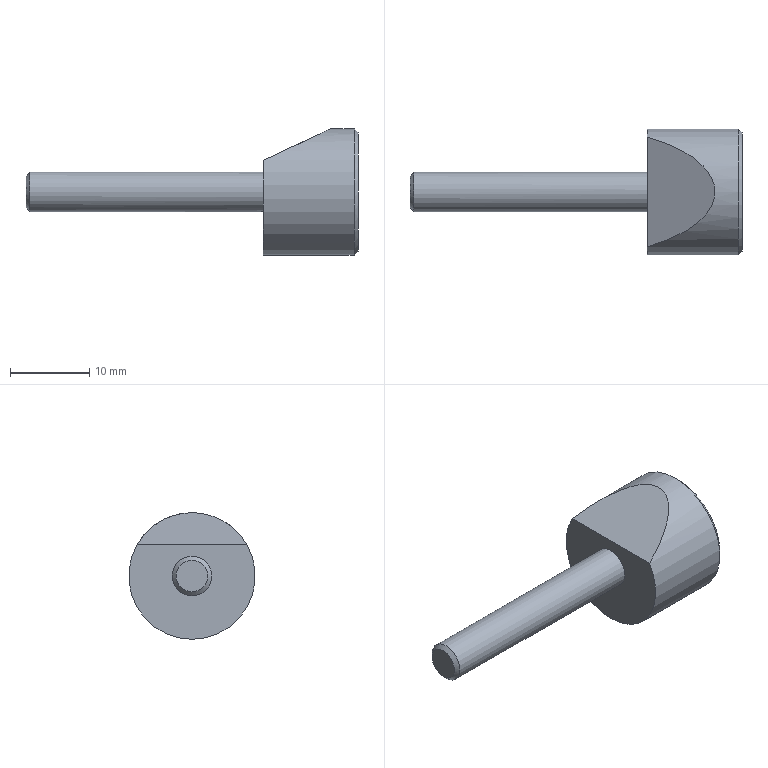Component | NX | LOCKING_SHAFT | 1 solid | 8 faces | box 42 x 16 x 16 mm | volume 2856 mm3 | plane 4 | cylinder 2 | cone 2 | commonest cylinder face diameters 16 x1 5 x1
STEP:
#1=CARTESIAN_POINT('',(0.,0.,0.));
#2=DIRECTION('',(0.,0.,1.));
#3=DIRECTION('',(1.,0.,0.));
#4=AXIS2_PLACEMENT_3D('',#1,#2,#3);
#5=CARTESIAN_POINT('',(109.666,163.398,144.15));
#6=VERTEX_POINT('',#5);
#7=CARTESIAN_POINT('',(109.666,170.327,156.15));
#8=VERTEX_POINT('',#7);
#9=CARTESIAN_POINT('',(109.666,163.398,152.15));
#10=DIRECTION('',(-1.,0.,0.));
#11=DIRECTION('',(0.,0.,-1.));
#12=AXIS2_PLACEMENT_3D('',#9,#10,#11);
#13=CIRCLE('',#12,8.);
#14=CARTESIAN_POINT('',(98.166,163.398,152.15));
#15=DIRECTION('',(1.,0.,0.));
#16=DIRECTION('',(0.,0.,1.));
#17=AXIS2_PLACEMENT_3D('',#14,#15,#16);
#18=CYLINDRICAL_SURFACE('',#17,8.);
#19=CARTESIAN_POINT('',(9.425,11.5));
#20=DIRECTION('',(-1.,0.));
#21=VECTOR('',#20,1.);
#22=LINE('',#19,#21);
#23=(GEOMETRIC_REPRESENTATION_CONTEXT(2)PARAMETRIC_REPRESENTATION_CONTEXT()REPRESENTATION_CONTEXT('',''));
#24=DEFINITIONAL_REPRESENTATION('',(#22),#23);
#25=PCURVE('',#18,#24);
#26=CARTESIAN_POINT('',(109.666,163.398,152.15));
#27=DIRECTION('',(-1.,0.,0.));
#28=DIRECTION('',(0.,0.,-1.));
#29=AXIS2_PLACEMENT_3D('',#26,#27,#28);
#30=CONICAL_SURFACE('',#29,8.,0.7854);
#31=CARTESIAN_POINT('',(0.,0.));
#32=DIRECTION('',(1.,0.));
#33=VECTOR('',#32,1.);
#34=LINE('',#31,#33);
#35=(GEOMETRIC_REPRESENTATION_CONTEXT(2)PARAMETRIC_REPRESENTATION_CONTEXT()REPRESENTATION_CONTEXT('',''));
#36=DEFINITIONAL_REPRESENTATION('',(#34),#35);
#37=PCURVE('',#30,#36);
#38=SURFACE_CURVE('',#13,(#25,#37),.PCURVE_S1.);
#39=EDGE_CURVE('',#6,#8,#38,.T.);
#40=ORIENTED_EDGE('',*,*,#39,.T.);
#41=CARTESIAN_POINT('',(98.166,170.327,156.15));
#42=VERTEX_POINT('',#41);
#43=CARTESIAN_POINT('',(98.166,170.327,156.15));
#44=CARTESIAN_POINT('',(109.666,170.327,156.15));
#45=B_SPLINE_CURVE_WITH_KNOTS('',1,(#43,#44),.UNSPECIFIED.,.F.,.F.,(2,2),(0.,11.5),.PIECEWISE_BEZIER_KNOTS.);
#46=CARTESIAN_POINT('',(5.236,0.));
#47=DIRECTION('',(0.,1.));
#48=VECTOR('',#47,1.);
#49=LINE('',#46,#48);
#50=(GEOMETRIC_REPRESENTATION_CONTEXT(2)PARAMETRIC_REPRESENTATION_CONTEXT()REPRESENTATION_CONTEXT('',''));
#51=DEFINITIONAL_REPRESENTATION('',(#49),#50);
#52=PCURVE('',#18,#51);
#53=CARTESIAN_POINT('',(11.519,0.));
#54=DIRECTION('',(0.,1.));
#55=VECTOR('',#54,1.);
#56=LINE('',#53,#55);
#57=(GEOMETRIC_REPRESENTATION_CONTEXT(2)PARAMETRIC_REPRESENTATION_CONTEXT()REPRESENTATION_CONTEXT('',''));
#58=DEFINITIONAL_REPRESENTATION('',(#56),#57);
#59=PCURVE('',#18,#58);
#60=SEAM_CURVE('',#45,(#52,#59),.PCURVE_S1.);
#61=EDGE_CURVE('',#42,#8,#60,.T.);
#62=ORIENTED_EDGE('',*,*,#61,.F.);
#63=CARTESIAN_POINT('',(98.166,156.47,156.15));
#64=VERTEX_POINT('',#63);
#65=CARTESIAN_POINT('',(89.588,163.398,152.15));
#66=DIRECTION('',(-0.4226,0.,0.9063));
#67=DIRECTION('',(0.9063,0.,0.4226));
#68=AXIS2_PLACEMENT_3D('',#65,#66,#67);
#69=ELLIPSE('',#68,18.93,8.);
#70=CARTESIAN_POINT('',(7.33,-0.));
#71=CARTESIAN_POINT('',(7.299,0.4715));
#72=CARTESIAN_POINT('',(7.235,1.388));
#73=CARTESIAN_POINT('',(7.14,2.674));
#74=CARTESIAN_POINT('',(7.045,3.857));
#75=CARTESIAN_POINT('',(6.95,4.928));
#76=CARTESIAN_POINT('',(6.854,5.876));
#77=CARTESIAN_POINT('',(6.759,6.694));
#78=CARTESIAN_POINT('',(6.664,7.373));
#79=CARTESIAN_POINT('',(6.569,7.908));
#80=CARTESIAN_POINT('',(6.474,8.293));
#81=CARTESIAN_POINT('',(6.378,8.526));
#82=CARTESIAN_POINT('',(6.283,8.604));
#83=CARTESIAN_POINT('',(6.188,8.526));
#84=CARTESIAN_POINT('',(6.093,8.293));
#85=CARTESIAN_POINT('',(5.998,7.908));
#86=CARTESIAN_POINT('',(5.902,7.373));
#87=CARTESIAN_POINT('',(5.807,6.694));
#88=CARTESIAN_POINT('',(5.712,5.876));
#89=CARTESIAN_POINT('',(5.617,4.928));
#90=CARTESIAN_POINT('',(5.522,3.857));
#91=CARTESIAN_POINT('',(5.426,2.674));
#92=CARTESIAN_POINT('',(5.331,1.388));
#93=CARTESIAN_POINT('',(5.268,0.4715));
#94=CARTESIAN_POINT('',(5.236,0.));
#95=B_SPLINE_CURVE_WITH_KNOTS('',3,(#70,#71,#72,#73,#74,#75,#76,#77,#78,#79,#80,#81,#82,#83,#84,#85,#86,#87,#88,#89,#90,#91,#92,#93,#94),.UNSPECIFIED.,.F.,.F.,(4,1,1,1,1,1,1,1,1,1,1,1,1,1,1,1,1,1,1,1,1,1,4),(5.236,5.331,5.426,5.522,5.617,5.712,5.807,5.902,5.998,6.093,6.188,6.283,6.378,6.474,6.569,6.664,6.759,6.854,6.95,7.045,7.14,7.235,7.33),.QUASI_UNIFORM_KNOTS.);
#96=(GEOMETRIC_REPRESENTATION_CONTEXT(2)PARAMETRIC_REPRESENTATION_CONTEXT()REPRESENTATION_CONTEXT('',''));
#97=DEFINITIONAL_REPRESENTATION('',(#95),#96);
#98=PCURVE('',#18,#97);
#99=CARTESIAN_POINT('',(98.166,133.398,156.15));
#100=DIRECTION('',(-0.4226,0.,0.9063));
#101=DIRECTION('',(-0.9063,0.,-0.4226));
#102=AXIS2_PLACEMENT_3D('',#99,#100,#101);
#103=PLANE('',#102);
#104=CARTESIAN_POINT('',(9.465,-30.));
#105=DIRECTION('',(-1.,0.));
#106=AXIS2_PLACEMENT_2D('',#104,#105);
#107=ELLIPSE('',#106,18.93,8.);
#108=(GEOMETRIC_REPRESENTATION_CONTEXT(2)PARAMETRIC_REPRESENTATION_CONTEXT()REPRESENTATION_CONTEXT('',''));
#109=DEFINITIONAL_REPRESENTATION('',(#107),#108);
#110=PCURVE('',#103,#109);
#111=SURFACE_CURVE('',#69,(#98,#110),.PCURVE_S1.);
#112=EDGE_CURVE('',#64,#42,#111,.T.);
#113=ORIENTED_EDGE('',*,*,#112,.F.);
#114=CARTESIAN_POINT('',(98.166,163.398,152.15));
#115=DIRECTION('',(-1.,0.,0.));
#116=DIRECTION('',(0.,-1.,0.));
#117=AXIS2_PLACEMENT_3D('',#114,#115,#116);
#118=CIRCLE('',#117,8.);
#119=CARTESIAN_POINT('',(14.137,0.));
#120=DIRECTION('',(-1.,0.));
#121=VECTOR('',#120,1.);
#122=LINE('',#119,#121);
#123=(GEOMETRIC_REPRESENTATION_CONTEXT(2)PARAMETRIC_REPRESENTATION_CONTEXT()REPRESENTATION_CONTEXT('',''));
#124=DEFINITIONAL_REPRESENTATION('',(#122),#123);
#125=PCURVE('',#18,#124);
#126=CARTESIAN_POINT('',(98.166,163.398,152.15));
#127=DIRECTION('',(-1.,0.,0.));
#128=DIRECTION('',(0.,0.,-1.));
#129=AXIS2_PLACEMENT_3D('',#126,#127,#128);
#130=PLANE('',#129);
#131=CARTESIAN_POINT('',(0.,0.));
#132=DIRECTION('',(0.,1.));
#133=AXIS2_PLACEMENT_2D('',#131,#132);
#134=CIRCLE('',#133,8.);
#135=(GEOMETRIC_REPRESENTATION_CONTEXT(2)PARAMETRIC_REPRESENTATION_CONTEXT()REPRESENTATION_CONTEXT('',''));
#136=DEFINITIONAL_REPRESENTATION('',(#134),#135);
#137=PCURVE('',#130,#136);
#138=SURFACE_CURVE('',#118,(#125,#137),.PCURVE_S1.);
#139=EDGE_CURVE('',#42,#64,#138,.T.);
#140=ORIENTED_EDGE('',*,*,#139,.F.);
#141=ORIENTED_EDGE('',*,*,#61,.T.);
#142=CARTESIAN_POINT('',(109.666,163.398,152.15));
#143=DIRECTION('',(-1.,0.,0.));
#144=DIRECTION('',(0.,0.,-1.));
#145=AXIS2_PLACEMENT_3D('',#142,#143,#144);
#146=CIRCLE('',#145,8.);
#147=CARTESIAN_POINT('',(15.708,11.5));
#148=DIRECTION('',(-1.,0.));
#149=VECTOR('',#148,1.);
#150=LINE('',#147,#149);
#151=(GEOMETRIC_REPRESENTATION_CONTEXT(2)PARAMETRIC_REPRESENTATION_CONTEXT()REPRESENTATION_CONTEXT('',''));
#152=DEFINITIONAL_REPRESENTATION('',(#150),#151);
#153=PCURVE('',#18,#152);
#154=CARTESIAN_POINT('',(0.,0.));
#155=DIRECTION('',(1.,-0.));
#156=VECTOR('',#155,1.);
#157=LINE('',#154,#156);
#158=(GEOMETRIC_REPRESENTATION_CONTEXT(2)PARAMETRIC_REPRESENTATION_CONTEXT()REPRESENTATION_CONTEXT('',''));
#159=DEFINITIONAL_REPRESENTATION('',(#157),#158);
#160=PCURVE('',#30,#159);
#161=SURFACE_CURVE('',#146,(#153,#160),.PCURVE_S1.);
#162=EDGE_CURVE('',#8,#6,#161,.T.);
#163=ORIENTED_EDGE('',*,*,#162,.T.);
#164=EDGE_LOOP('',(#40,#62,#113,#140,#141,#163));
#165=FACE_BOUND('',#164,.T.);
#166=ADVANCED_FACE('',(#165),#18,.T.);
#167=CARTESIAN_POINT('',(98.166,160.898,152.15));
#168=VERTEX_POINT('',#167);
#169=CARTESIAN_POINT('',(98.166,163.398,152.15));
#170=DIRECTION('',(-1.,0.,0.));
#171=DIRECTION('',(0.,-1.,0.));
#172=AXIS2_PLACEMENT_3D('',#169,#170,#171);
#173=CIRCLE('',#172,2.5);
#174=CARTESIAN_POINT('',(0.,0.));
#175=DIRECTION('',(0.,1.));
#176=AXIS2_PLACEMENT_2D('',#174,#175);
#177=CIRCLE('',#176,2.5);
#178=(GEOMETRIC_REPRESENTATION_CONTEXT(2)PARAMETRIC_REPRESENTATION_CONTEXT()REPRESENTATION_CONTEXT('',''));
#179=DEFINITIONAL_REPRESENTATION('',(#177),#178);
#180=PCURVE('',#130,#179);
#181=CARTESIAN_POINT('',(68.166,163.398,152.15));
#182=DIRECTION('',(1.,0.,0.));
#183=DIRECTION('',(0.,0.,1.));
#184=AXIS2_PLACEMENT_3D('',#181,#182,#183);
#185=CYLINDRICAL_SURFACE('',#184,2.5);
#186=CARTESIAN_POINT('',(7.854,30.));
#187=DIRECTION('',(-1.,0.));
#188=VECTOR('',#187,1.);
#189=LINE('',#186,#188);
#190=(GEOMETRIC_REPRESENTATION_CONTEXT(2)PARAMETRIC_REPRESENTATION_CONTEXT()REPRESENTATION_CONTEXT('',''));
#191=DEFINITIONAL_REPRESENTATION('',(#189),#190);
#192=PCURVE('',#185,#191);
#193=SURFACE_CURVE('',#173,(#180,#192),.PCURVE_S1.);
#194=EDGE_CURVE('',#168,#168,#193,.T.);
#195=ORIENTED_EDGE('',*,*,#194,.F.);
#196=EDGE_LOOP('',(#195));
#197=FACE_BOUND('',#196,.T.);
#198=ORIENTED_EDGE('',*,*,#139,.T.);
#199=CARTESIAN_POINT('',(98.166,133.398,156.15));
#200=DIRECTION('',(0.,1.,0.));
#201=VECTOR('',#200,1.);
#202=LINE('',#199,#201);
#203=CARTESIAN_POINT('',(-4.,30.));
#204=DIRECTION('',(0.,-1.));
#205=VECTOR('',#204,1.);
#206=LINE('',#203,#205);
#207=(GEOMETRIC_REPRESENTATION_CONTEXT(2)PARAMETRIC_REPRESENTATION_CONTEXT()REPRESENTATION_CONTEXT('',''));
#208=DEFINITIONAL_REPRESENTATION('',(#206),#207);
#209=PCURVE('',#130,#208);
#210=CARTESIAN_POINT('',(0.,0.));
#211=DIRECTION('',(0.,-1.));
#212=VECTOR('',#211,1.);
#213=LINE('',#210,#212);
#214=(GEOMETRIC_REPRESENTATION_CONTEXT(2)PARAMETRIC_REPRESENTATION_CONTEXT()REPRESENTATION_CONTEXT('',''));
#215=DEFINITIONAL_REPRESENTATION('',(#213),#214);
#216=PCURVE('',#103,#215);
#217=SURFACE_CURVE('',#202,(#209,#216),.PCURVE_S1.);
#218=EDGE_CURVE('',#64,#42,#217,.T.);
#219=ORIENTED_EDGE('',*,*,#218,.T.);
#220=EDGE_LOOP('',(#198,#219));
#221=FACE_BOUND('',#220,.T.);
#222=ADVANCED_FACE('',(#197,#221),#130,.T.);
#223=CARTESIAN_POINT('',(110.166,163.398,144.65));
#224=VERTEX_POINT('',#223);
#225=CARTESIAN_POINT('',(110.166,163.398,152.15));
#226=DIRECTION('',(1.,0.,0.));
#227=DIRECTION('',(0.,0.,-1.));
#228=AXIS2_PLACEMENT_3D('',#225,#226,#227);
#229=CIRCLE('',#228,7.5);
#230=CARTESIAN_POINT('',(110.166,163.398,152.15));
#231=DIRECTION('',(-1.,0.,0.));
#232=DIRECTION('',(0.,0.,-1.));
#233=AXIS2_PLACEMENT_3D('',#230,#231,#232);
#234=PLANE('',#233);
#235=CARTESIAN_POINT('',(7.5,0.));
#236=CARTESIAN_POINT('',(7.5,-12.99));
#237=CARTESIAN_POINT('',(-3.75,-6.495));
#238=CARTESIAN_POINT('',(-15.,-0.));
#239=CARTESIAN_POINT('',(-3.75,6.495));
#240=CARTESIAN_POINT('',(7.5,12.99));
#241=CARTESIAN_POINT('',(7.5,0.));
#242=(BOUNDED_CURVE()B_SPLINE_CURVE(2,(#235,#236,#237,#238,#239,#240,#241),.UNSPECIFIED.,.T.,.F.)B_SPLINE_CURVE_WITH_KNOTS((1,2,2,2,2,1),(-2.094,0.,2.094,4.189,6.283,8.378),.UNSPECIFIED.)CURVE()GEOMETRIC_REPRESENTATION_ITEM()RATIONAL_B_SPLINE_CURVE((1.,0.5,1.,0.5,1.,0.5,1.))REPRESENTATION_ITEM(''));
#243=(GEOMETRIC_REPRESENTATION_CONTEXT(2)PARAMETRIC_REPRESENTATION_CONTEXT()REPRESENTATION_CONTEXT('',''));
#244=DEFINITIONAL_REPRESENTATION('',(#242),#243);
#245=PCURVE('',#234,#244);
#246=CARTESIAN_POINT('',(6.283,-0.5));
#247=DIRECTION('',(-1.,0.));
#248=VECTOR('',#247,1.);
#249=LINE('',#246,#248);
#250=(GEOMETRIC_REPRESENTATION_CONTEXT(2)PARAMETRIC_REPRESENTATION_CONTEXT()REPRESENTATION_CONTEXT('',''));
#251=DEFINITIONAL_REPRESENTATION('',(#249),#250);
#252=PCURVE('',#30,#251);
#253=SURFACE_CURVE('',#229,(#245,#252),.PCURVE_S1.);
#254=EDGE_CURVE('',#224,#224,#253,.T.);
#255=ORIENTED_EDGE('',*,*,#254,.T.);
#256=EDGE_LOOP('',(#255));
#257=FACE_BOUND('',#256,.T.);
#258=ADVANCED_FACE('',(#257),#234,.F.);
#259=CARTESIAN_POINT('',(68.666,163.398,149.65));
#260=VERTEX_POINT('',#259);
#261=CARTESIAN_POINT('',(68.666,160.898,152.15));
#262=VERTEX_POINT('',#261);
#263=CARTESIAN_POINT('',(68.666,163.398,152.15));
#264=DIRECTION('',(1.,0.,0.));
#265=DIRECTION('',(0.,0.,-1.));
#266=AXIS2_PLACEMENT_3D('',#263,#264,#265);
#267=CIRCLE('',#266,2.5);
#268=CARTESIAN_POINT('',(3.142,0.5));
#269=DIRECTION('',(1.,0.));
#270=VECTOR('',#269,1.);
#271=LINE('',#268,#270);
#272=(GEOMETRIC_REPRESENTATION_CONTEXT(2)PARAMETRIC_REPRESENTATION_CONTEXT()REPRESENTATION_CONTEXT('',''));
#273=DEFINITIONAL_REPRESENTATION('',(#271),#272);
#274=PCURVE('',#185,#273);
#275=CARTESIAN_POINT('',(68.166,163.398,152.15));
#276=DIRECTION('',(1.,0.,0.));
#277=DIRECTION('',(0.,0.,1.));
#278=AXIS2_PLACEMENT_3D('',#275,#276,#277);
#279=CONICAL_SURFACE('',#278,2.,0.7854);
#280=CARTESIAN_POINT('',(3.142,0.5));
#281=DIRECTION('',(1.,0.));
#282=VECTOR('',#281,1.);
#283=LINE('',#280,#282);
#284=(GEOMETRIC_REPRESENTATION_CONTEXT(2)PARAMETRIC_REPRESENTATION_CONTEXT()REPRESENTATION_CONTEXT('',''));
#285=DEFINITIONAL_REPRESENTATION('',(#283),#284);
#286=PCURVE('',#279,#285);
#287=SURFACE_CURVE('',#267,(#274,#286),.PCURVE_S1.);
#288=EDGE_CURVE('',#260,#262,#287,.T.);
#289=ORIENTED_EDGE('',*,*,#288,.T.);
#290=CARTESIAN_POINT('',(68.666,160.898,152.15));
#291=CARTESIAN_POINT('',(98.166,160.898,152.15));
#292=B_SPLINE_CURVE_WITH_KNOTS('',1,(#290,#291),.UNSPECIFIED.,.F.,.F.,(2,2),(0.5,30.),.PIECEWISE_BEZIER_KNOTS.);
#293=CARTESIAN_POINT('',(7.854,0.));
#294=DIRECTION('',(0.,1.));
#295=VECTOR('',#294,1.);
#296=LINE('',#293,#295);
#297=(GEOMETRIC_REPRESENTATION_CONTEXT(2)PARAMETRIC_REPRESENTATION_CONTEXT()REPRESENTATION_CONTEXT('',''));
#298=DEFINITIONAL_REPRESENTATION('',(#296),#297);
#299=PCURVE('',#185,#298);
#300=CARTESIAN_POINT('',(1.571,0.));
#301=DIRECTION('',(0.,1.));
#302=VECTOR('',#301,1.);
#303=LINE('',#300,#302);
#304=(GEOMETRIC_REPRESENTATION_CONTEXT(2)PARAMETRIC_REPRESENTATION_CONTEXT()REPRESENTATION_CONTEXT('',''));
#305=DEFINITIONAL_REPRESENTATION('',(#303),#304);
#306=PCURVE('',#185,#305);
#307=SEAM_CURVE('',#292,(#299,#306),.PCURVE_S1.);
#308=EDGE_CURVE('',#262,#168,#307,.T.);
#309=ORIENTED_EDGE('',*,*,#308,.T.);
#310=ORIENTED_EDGE('',*,*,#194,.T.);
#311=ORIENTED_EDGE('',*,*,#308,.F.);
#312=CARTESIAN_POINT('',(68.666,163.398,152.15));
#313=DIRECTION('',(1.,0.,0.));
#314=DIRECTION('',(0.,0.,-1.));
#315=AXIS2_PLACEMENT_3D('',#312,#313,#314);
#316=CIRCLE('',#315,2.5);
#317=CARTESIAN_POINT('',(-3.142,0.5));
#318=DIRECTION('',(1.,0.));
#319=VECTOR('',#318,1.);
#320=LINE('',#317,#319);
#321=(GEOMETRIC_REPRESENTATION_CONTEXT(2)PARAMETRIC_REPRESENTATION_CONTEXT()REPRESENTATION_CONTEXT('',''));
#322=DEFINITIONAL_REPRESENTATION('',(#320),#321);
#323=PCURVE('',#185,#322);
#324=CARTESIAN_POINT('',(3.142,0.5));
#325=DIRECTION('',(1.,0.));
#326=VECTOR('',#325,1.);
#327=LINE('',#324,#326);
#328=(GEOMETRIC_REPRESENTATION_CONTEXT(2)PARAMETRIC_REPRESENTATION_CONTEXT()REPRESENTATION_CONTEXT('',''));
#329=DEFINITIONAL_REPRESENTATION('',(#327),#328);
#330=PCURVE('',#279,#329);
#331=SURFACE_CURVE('',#316,(#323,#330),.PCURVE_S1.);
#332=EDGE_CURVE('',#262,#260,#331,.T.);
#333=ORIENTED_EDGE('',*,*,#332,.T.);
#334=EDGE_LOOP('',(#289,#309,#310,#311,#333));
#335=FACE_BOUND('',#334,.T.);
#336=ADVANCED_FACE('',(#335),#185,.T.);
#337=CARTESIAN_POINT('',(68.166,163.398,150.15));
#338=VERTEX_POINT('',#337);
#339=CARTESIAN_POINT('',(68.166,163.398,152.15));
#340=DIRECTION('',(-1.,0.,0.));
#341=DIRECTION('',(0.,0.,-1.));
#342=AXIS2_PLACEMENT_3D('',#339,#340,#341);
#343=CIRCLE('',#342,2.);
#344=CARTESIAN_POINT('',(68.166,163.398,152.15));
#345=DIRECTION('',(-1.,0.,0.));
#346=DIRECTION('',(0.,0.,-1.));
#347=AXIS2_PLACEMENT_3D('',#344,#345,#346);
#348=PLANE('',#347);
#349=CARTESIAN_POINT('',(0.,0.));
#350=DIRECTION('',(1.,0.));
#351=AXIS2_PLACEMENT_2D('',#349,#350);
#352=CIRCLE('',#351,2.);
#353=(GEOMETRIC_REPRESENTATION_CONTEXT(2)PARAMETRIC_REPRESENTATION_CONTEXT()REPRESENTATION_CONTEXT('',''));
#354=DEFINITIONAL_REPRESENTATION('',(#352),#353);
#355=PCURVE('',#348,#354);
#356=CARTESIAN_POINT('',(9.425,0.));
#357=DIRECTION('',(-1.,0.));
#358=VECTOR('',#357,1.);
#359=LINE('',#356,#358);
#360=(GEOMETRIC_REPRESENTATION_CONTEXT(2)PARAMETRIC_REPRESENTATION_CONTEXT()REPRESENTATION_CONTEXT('',''));
#361=DEFINITIONAL_REPRESENTATION('',(#359),#360);
#362=PCURVE('',#279,#361);
#363=SURFACE_CURVE('',#343,(#355,#362),.PCURVE_S1.);
#364=EDGE_CURVE('',#338,#338,#363,.T.);
#365=ORIENTED_EDGE('',*,*,#364,.T.);
#366=EDGE_LOOP('',(#365));
#367=FACE_BOUND('',#366,.T.);
#368=ADVANCED_FACE('',(#367),#348,.T.);
#369=ORIENTED_EDGE('',*,*,#112,.T.);
#370=ORIENTED_EDGE('',*,*,#218,.F.);
#371=EDGE_LOOP('',(#369,#370));
#372=FACE_BOUND('',#371,.T.);
#373=ADVANCED_FACE('',(#372),#103,.T.);
#374=ORIENTED_EDGE('',*,*,#254,.F.);
#375=CARTESIAN_POINT('',(110.166,163.398,144.65));
#376=CARTESIAN_POINT('',(109.666,163.398,144.15));
#377=B_SPLINE_CURVE_WITH_KNOTS('',1,(#375,#376),.UNSPECIFIED.,.F.,.F.,(2,2),(-0.7071,0.),.PIECEWISE_BEZIER_KNOTS.);
#378=CARTESIAN_POINT('',(6.283,0.));
#379=DIRECTION('',(0.,1.));
#380=VECTOR('',#379,1.);
#381=LINE('',#378,#380);
#382=(GEOMETRIC_REPRESENTATION_CONTEXT(2)PARAMETRIC_REPRESENTATION_CONTEXT()REPRESENTATION_CONTEXT('',''));
#383=DEFINITIONAL_REPRESENTATION('',(#381),#382);
#384=PCURVE('',#30,#383);
#385=CARTESIAN_POINT('',(0.,0.));
#386=DIRECTION('',(0.,1.));
#387=VECTOR('',#386,1.);
#388=LINE('',#385,#387);
#389=(GEOMETRIC_REPRESENTATION_CONTEXT(2)PARAMETRIC_REPRESENTATION_CONTEXT()REPRESENTATION_CONTEXT('',''));
#390=DEFINITIONAL_REPRESENTATION('',(#388),#389);
#391=PCURVE('',#30,#390);
#392=SEAM_CURVE('',#377,(#384,#391),.PCURVE_S1.);
#393=EDGE_CURVE('',#224,#6,#392,.T.);
#394=ORIENTED_EDGE('',*,*,#393,.T.);
#395=ORIENTED_EDGE('',*,*,#162,.F.);
#396=ORIENTED_EDGE('',*,*,#39,.F.);
#397=ORIENTED_EDGE('',*,*,#393,.F.);
#398=EDGE_LOOP('',(#374,#394,#395,#396,#397));
#399=FACE_BOUND('',#398,.T.);
#400=ADVANCED_FACE('',(#399),#30,.T.);
#401=ORIENTED_EDGE('',*,*,#288,.F.);
#402=CARTESIAN_POINT('',(68.166,163.398,150.15));
#403=CARTESIAN_POINT('',(68.666,163.398,149.65));
#404=B_SPLINE_CURVE_WITH_KNOTS('',1,(#402,#403),.UNSPECIFIED.,.F.,.F.,(2,2),(0.,0.7071),.PIECEWISE_BEZIER_KNOTS.);
#405=CARTESIAN_POINT('',(3.142,0.));
#406=DIRECTION('',(0.,1.));
#407=VECTOR('',#406,1.);
#408=LINE('',#405,#407);
#409=(GEOMETRIC_REPRESENTATION_CONTEXT(2)PARAMETRIC_REPRESENTATION_CONTEXT()REPRESENTATION_CONTEXT('',''));
#410=DEFINITIONAL_REPRESENTATION('',(#408),#409);
#411=PCURVE('',#279,#410);
#412=CARTESIAN_POINT('',(9.425,0.));
#413=DIRECTION('',(0.,1.));
#414=VECTOR('',#413,1.);
#415=LINE('',#412,#414);
#416=(GEOMETRIC_REPRESENTATION_CONTEXT(2)PARAMETRIC_REPRESENTATION_CONTEXT()REPRESENTATION_CONTEXT('',''));
#417=DEFINITIONAL_REPRESENTATION('',(#415),#416);
#418=PCURVE('',#279,#417);
#419=SEAM_CURVE('',#404,(#411,#418),.PCURVE_S1.);
#420=EDGE_CURVE('',#338,#260,#419,.T.);
#421=ORIENTED_EDGE('',*,*,#420,.F.);
#422=ORIENTED_EDGE('',*,*,#364,.F.);
#423=ORIENTED_EDGE('',*,*,#420,.T.);
#424=ORIENTED_EDGE('',*,*,#332,.F.);
#425=EDGE_LOOP('',(#401,#421,#422,#423,#424));
#426=FACE_BOUND('',#425,.T.);
#427=ADVANCED_FACE('',(#426),#279,.T.);
#428=CLOSED_SHELL('',(#166,#222,#258,#336,#368,#373,#400,#427));
#429=MANIFOLD_SOLID_BREP('',#428);
#430=(LENGTH_UNIT()NAMED_UNIT(*)SI_UNIT(.MILLI.,.METRE.));
#431=UNCERTAINTY_MEASURE_WITH_UNIT(LENGTH_MEASURE(0.000005),#430,'','');
#432=(NAMED_UNIT(*)PLANE_ANGLE_UNIT()SI_UNIT($,.RADIAN.));
#433=(NAMED_UNIT(*)SI_UNIT($,.STERADIAN.)SOLID_ANGLE_UNIT());
#434=(GEOMETRIC_REPRESENTATION_CONTEXT(3)GLOBAL_UNCERTAINTY_ASSIGNED_CONTEXT((#431))GLOBAL_UNIT_ASSIGNED_CONTEXT((#430,#432,#433))REPRESENTATION_CONTEXT('',''));
#435=ADVANCED_BREP_SHAPE_REPRESENTATION('',(#4,#429),#434);